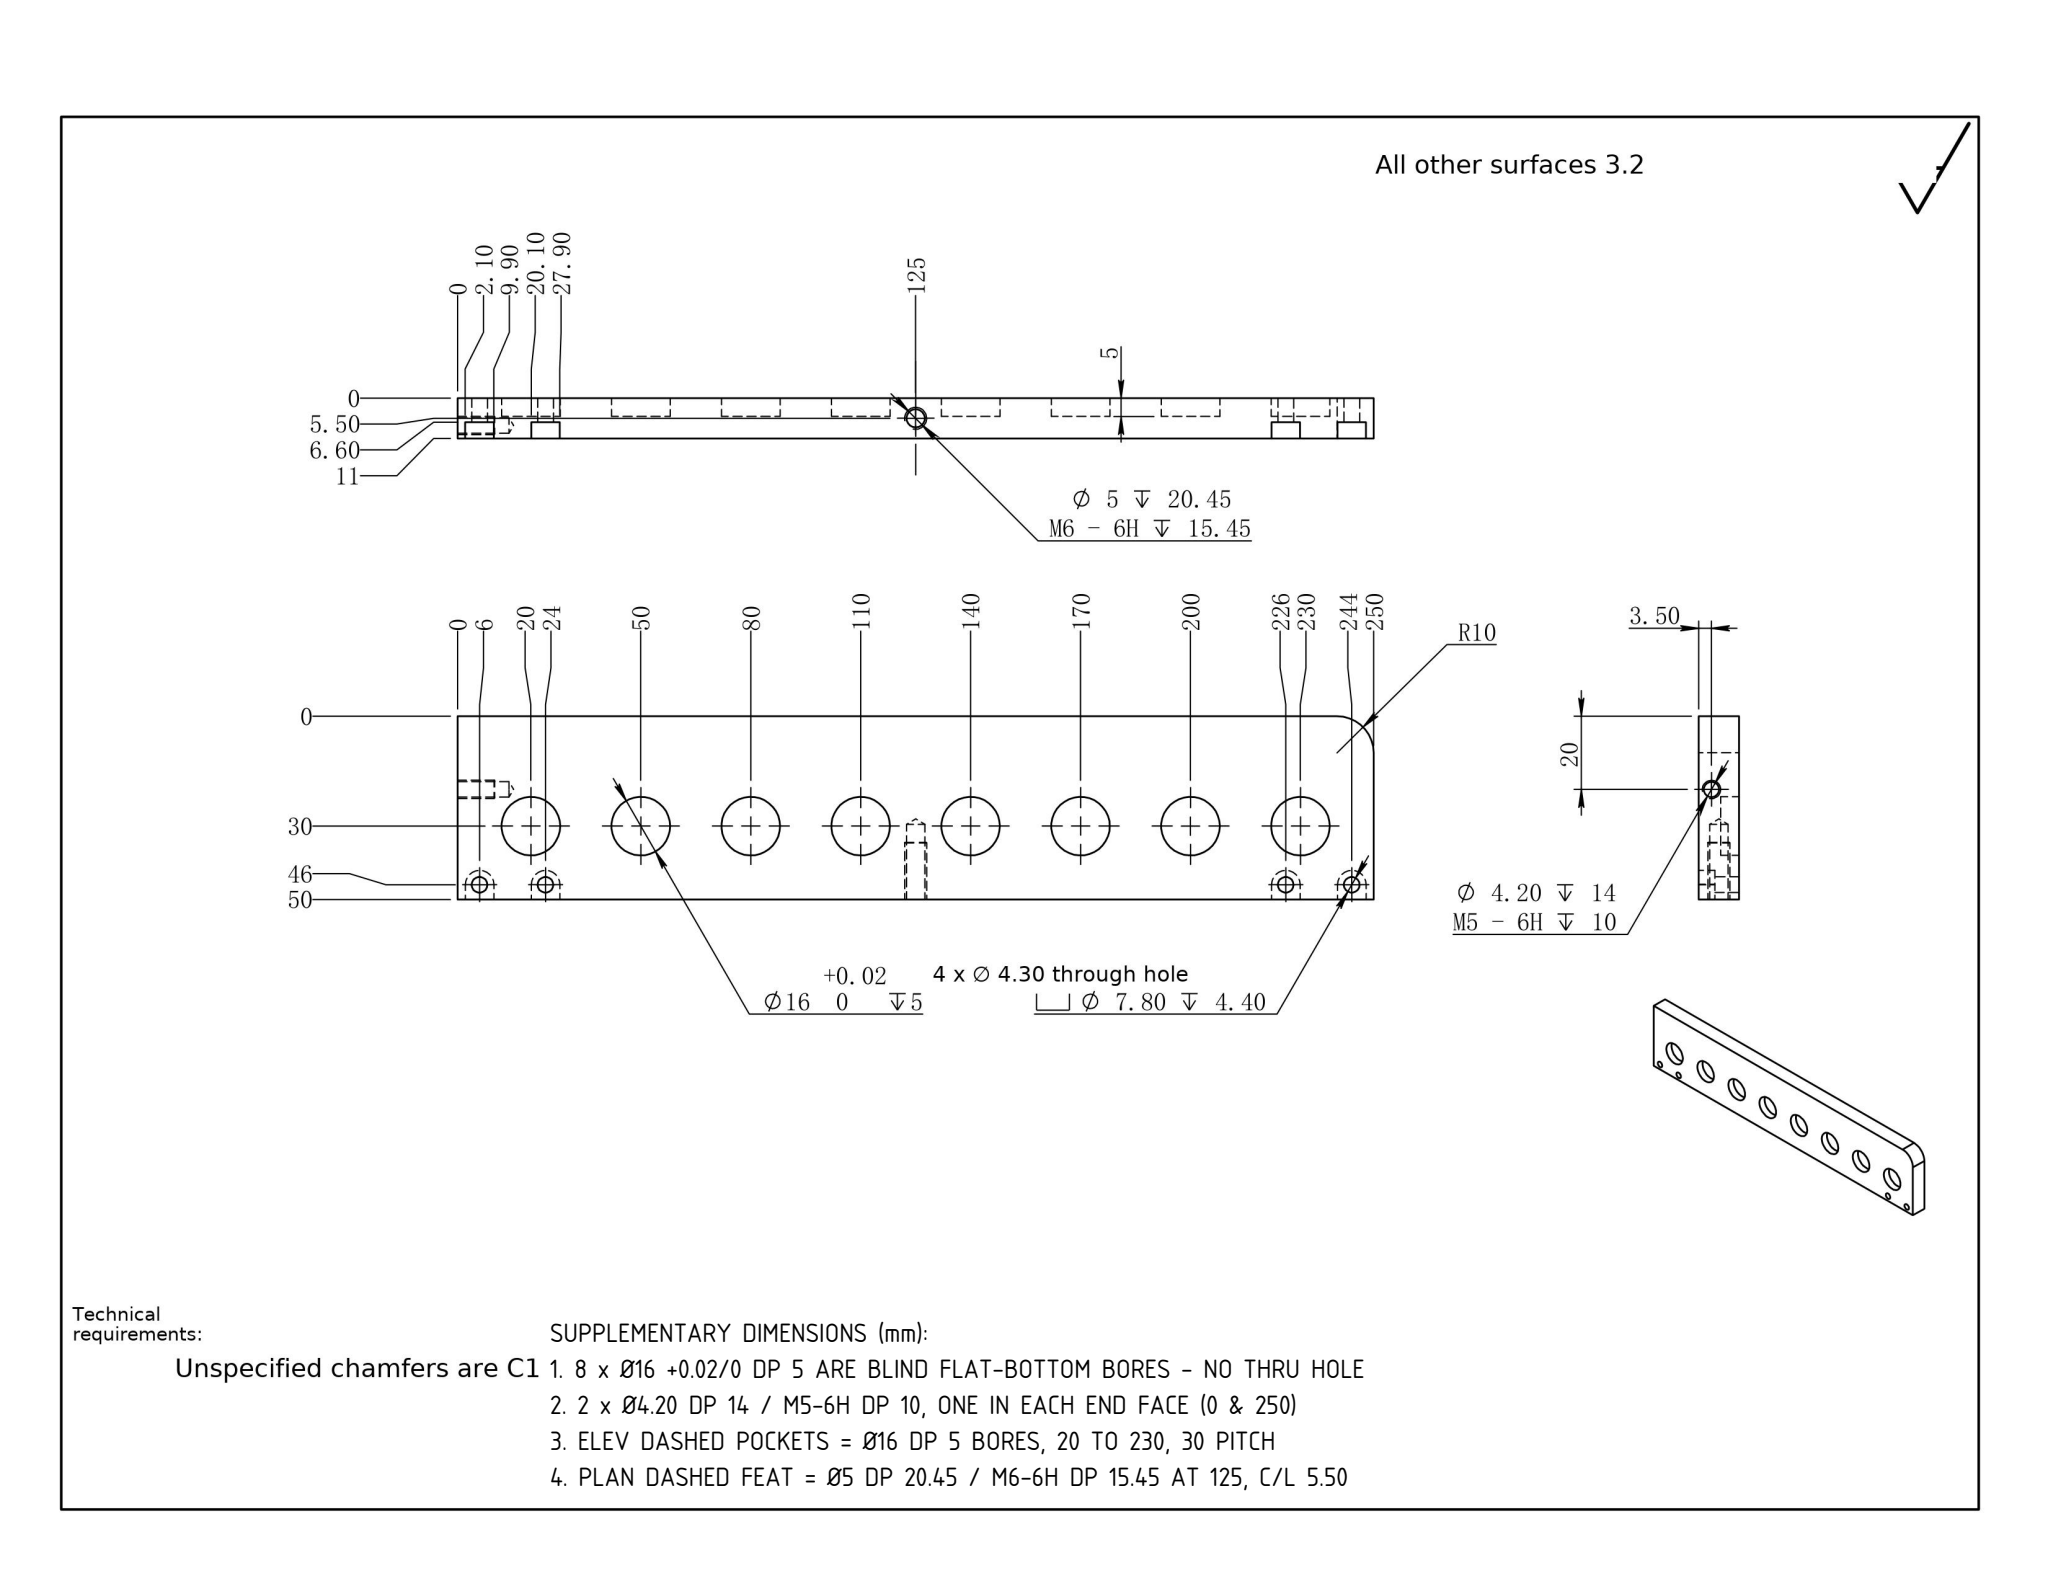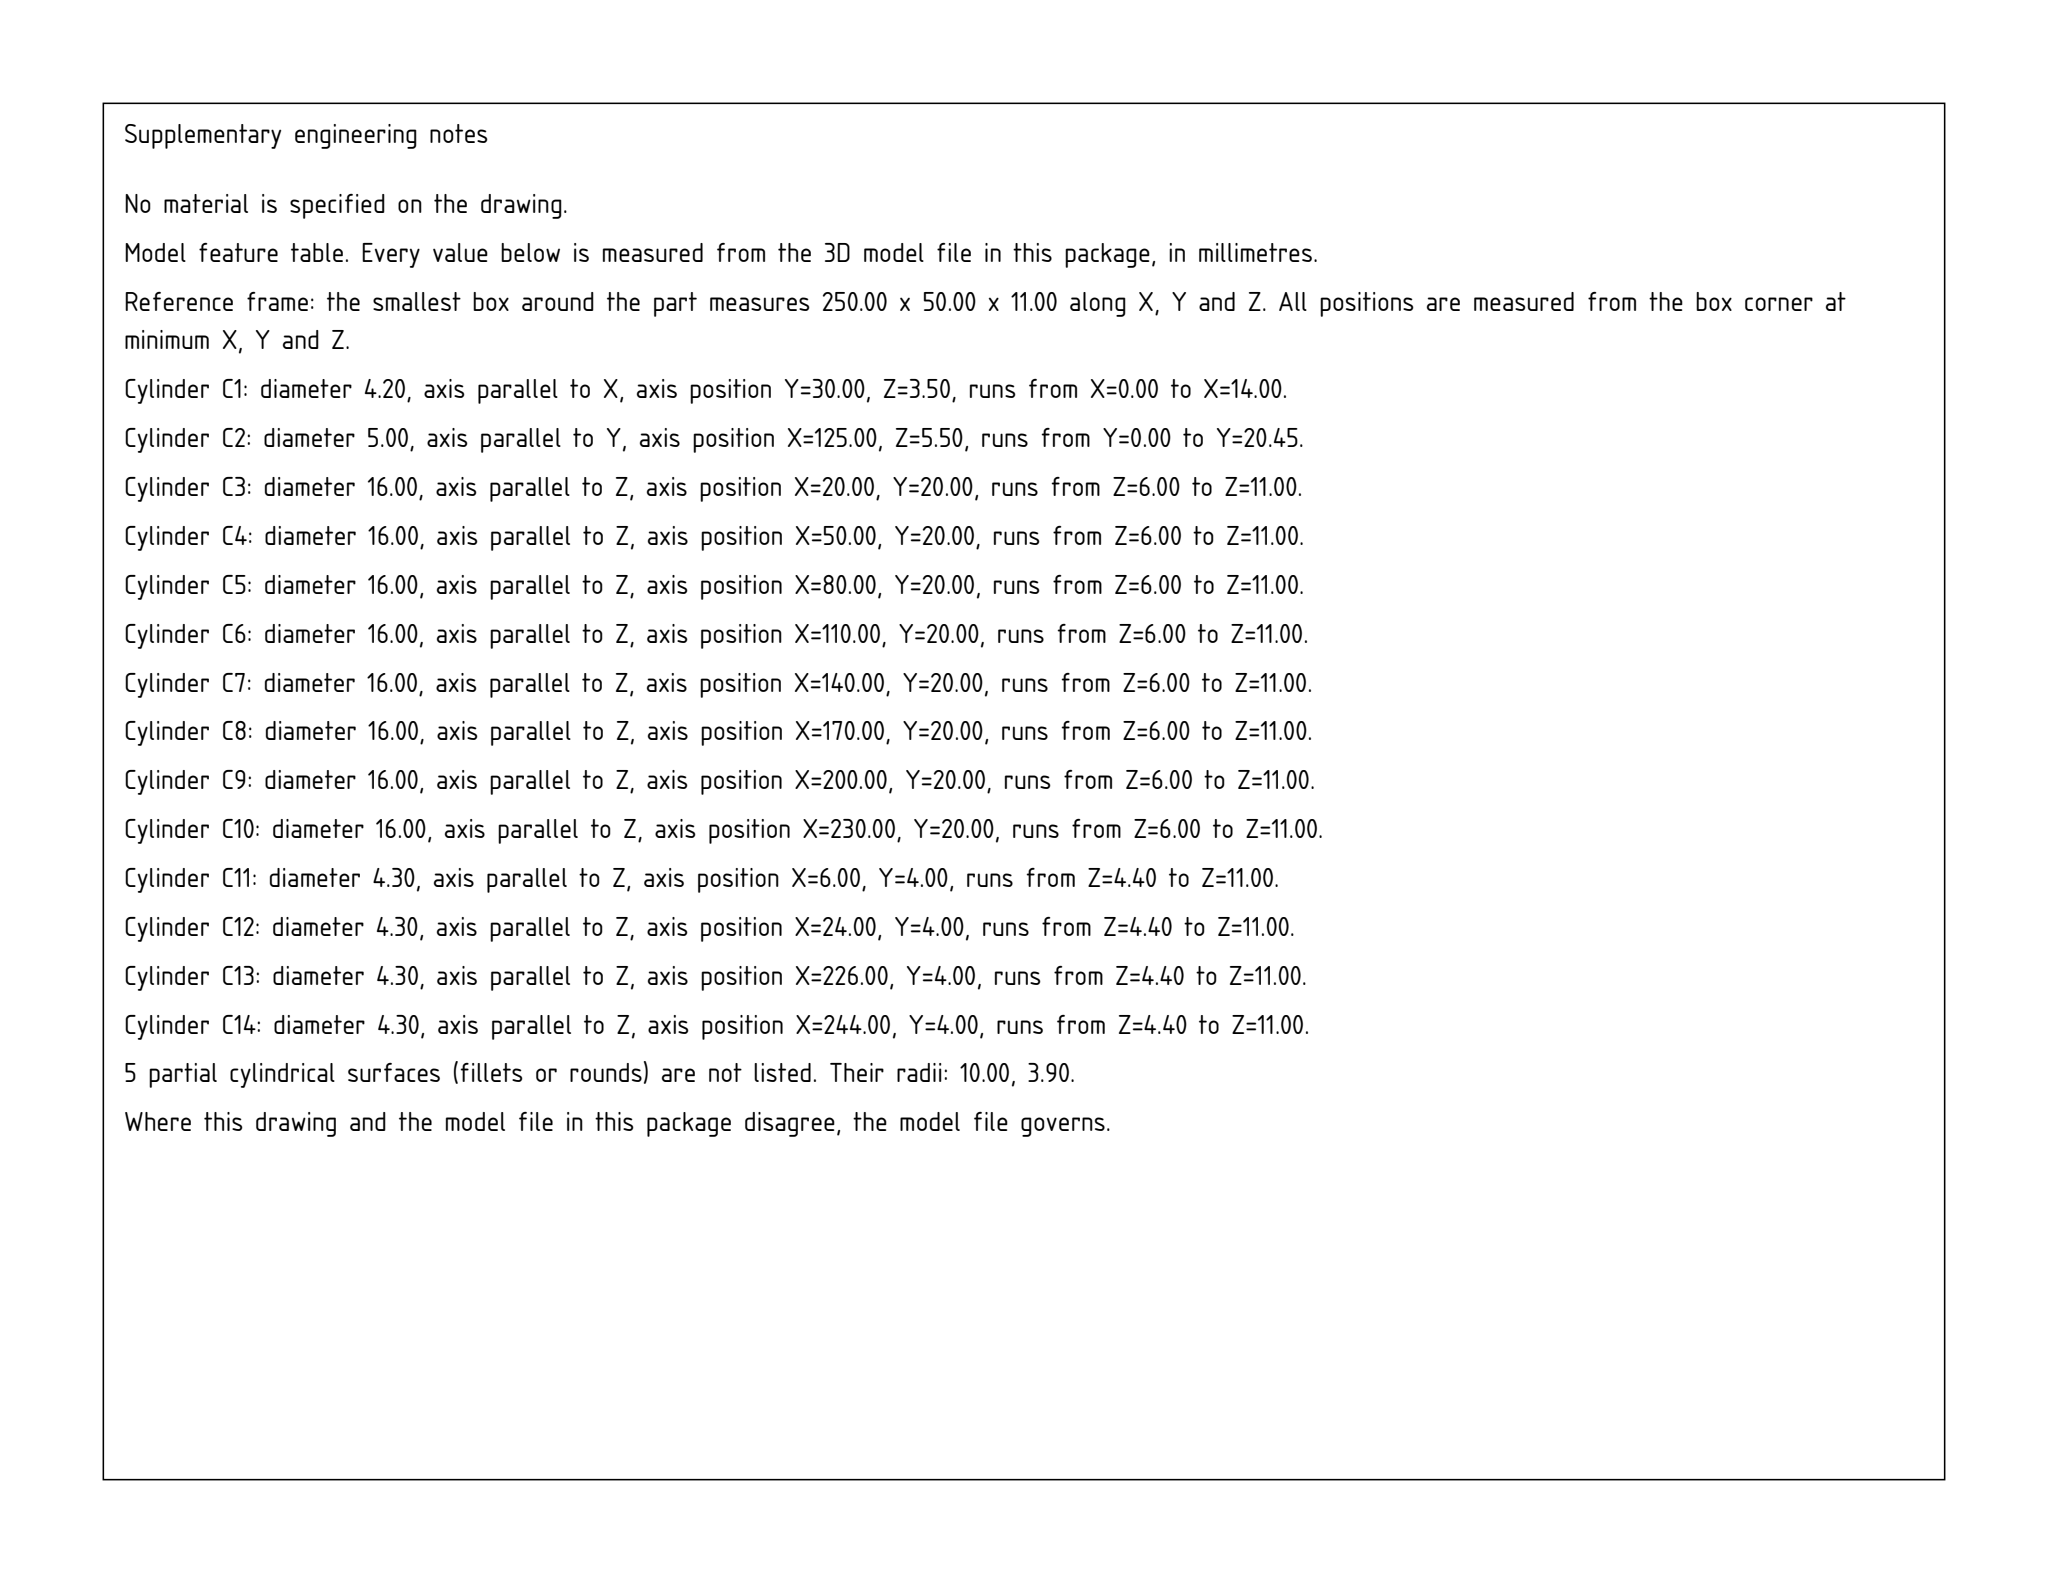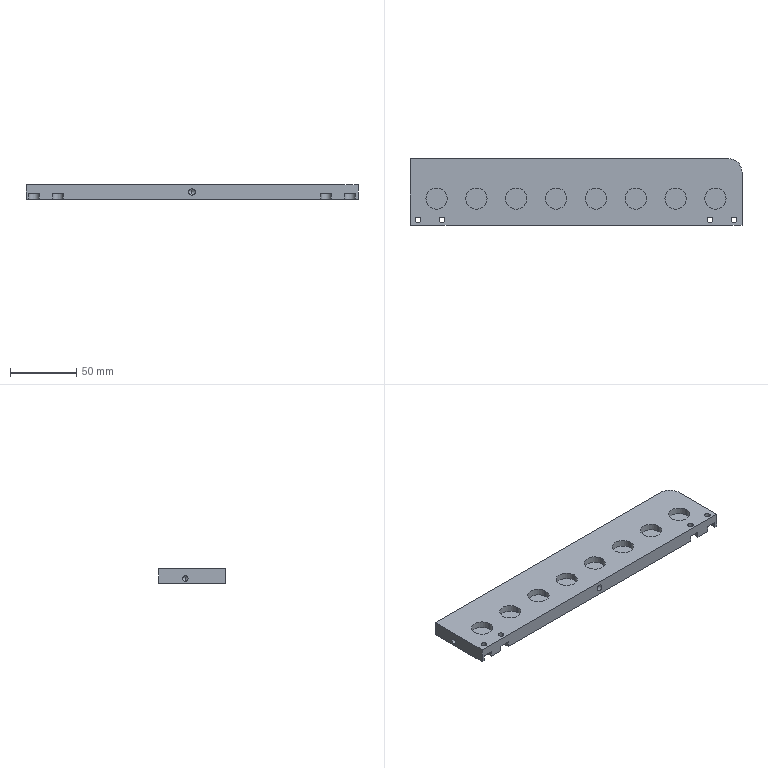Part | SolidWorks | mm | 1 solid | 63 faces | box 250 x 50 x 11 mm | volume 127257 mm3 | cylinder 33 | plane 26 | cone 4 | commonest cylinder face diameters 16 x16 4.3 x8 7.8 x4 4.2 x2 5 x2 20 x1
build123d program:
from build123d import *

# Parameters (mm, degrees)
SKETCH1_W                                       = 250
SKETCH1_H                                       = 50
BOSS_EXTRUDE1_DEPTH                             = 5.5
SKETCH2_R                                       = 8
CUT_EXTRUDE1_DEPTH                              = 5
LPATTERN1_COUNT                                 = 8
LPATTERN1_PITCH                                 = 30
FILLET4_R                                       = 10
M4_HEX_SOCKET_HEAD_CAP_SCREW_CBORE2_D           = 4.3
M4_HEX_SOCKET_HEAD_CAP_SCREW_CBORE2_CBORE_D     = 7.8
M4_HEX_SOCKET_HEAD_CAP_SCREW_CBORE2_CBORE_DEPTH = 4.4
CUT_EXTRUDE3_DEPTH                              = 128.646
M6_TAPPED_HOLE1_D                               = 5
M6_TAPPED_HOLE1_DEPTH                           = 20.45
M6_TAPPED_HOLE1_TIP                             = 1.502
M5_TAPPED_HOLE1_D                               = 4.2
M5_TAPPED_HOLE1_DEPTH                           = 14
M5_TAPPED_HOLE1_TIP                             = 1.262


with BuildPart() as part:
    # Sketch1 → Boss-Extrude1 (new, symmetric)
    with BuildSketch(Plane.XY):
        Rectangle(SKETCH1_W, SKETCH1_H)
    extrude(amount=BOSS_EXTRUDE1_DEPTH, both=True)

    # Sketch2 → Cut-Extrude1 (cut)
    with BuildSketch(Plane.XY.offset(5.5)):
        with Locations((105, -5)):
            Circle(SKETCH2_R)
    cut_extrude1 = extrude(amount=-CUT_EXTRUDE1_DEPTH, mode=Mode.SUBTRACT)

    # LPattern1: Cut-Extrude1 ×8
    with Locations(*[(-i * LPATTERN1_PITCH, 0, 0) for i in range(1, LPATTERN1_COUNT)]):
        add(cut_extrude1, mode=Mode.SUBTRACT)

    # Fillet4
    fillet4_edges = [part.edges().sort_by_distance(p)[0] for p in [
        (125, 25, 0),
    ]]
    fillet(fillet4_edges, radius=FILLET4_R)

    # M4 Hex Socket Head Cap Screw CBORE2 (through all)
    with Locations(Plane(origin=(0, 0, -5.5), x_dir=(-1, 0, 0), z_dir=(0, 0, -1))):
        with Locations((101, -21), (119, -21), (-119, -21), (-101, -21)):
            CounterBoreHole(M4_HEX_SOCKET_HEAD_CAP_SCREW_CBORE2_D / 2, M4_HEX_SOCKET_HEAD_CAP_SCREW_CBORE2_CBORE_D / 2, M4_HEX_SOCKET_HEAD_CAP_SCREW_CBORE2_CBORE_DEPTH)

    # Sketch8 → Cut-Extrude3 (cut, through all)
    with BuildSketch(Plane(origin=(0, 0, -1.1), x_dir=(-1, 0, 0), z_dir=(0, 0, -1))):
        with BuildLine():
            Line((-115.1, -21), (-115.1, -25))
            ThreePointArc((-115.1, -25), (-119, -28.9), (-122.9, -25))
            Line((-122.9, -25), (-122.9, -21))
            ThreePointArc((-122.9, -21), (-119, -17.1), (-115.1, -21))
        make_face()
        with BuildLine():
            Line((-97.1, -21), (-97.1, -25))
            ThreePointArc((-97.1, -25), (-101, -28.9), (-104.9, -25))
            Line((-104.9, -25), (-104.9, -21))
            ThreePointArc((-104.9, -21), (-101, -17.1), (-97.1, -21))
        make_face()
        with BuildLine():
            Line((104.9, -21), (104.9, -25))
            ThreePointArc((104.9, -25), (101, -28.9), (97.1, -25))
            Line((97.1, -25), (97.1, -21))
            ThreePointArc((97.1, -21), (101, -17.1), (104.9, -21))
        make_face()
        with BuildLine():
            Line((122.9, -21), (122.9, -25))
            ThreePointArc((122.9, -25), (119, -28.9), (115.1, -25))
            Line((115.1, -25), (115.1, -21))
            ThreePointArc((115.1, -21), (119, -17.1), (122.9, -21))
        make_face()
    extrude(amount=CUT_EXTRUDE3_DEPTH, mode=Mode.SUBTRACT)

    # M6 Tapped Hole1
    with Locations(Plane(origin=(0, -25, 0), x_dir=(-1, 0, 0), z_dir=(0, -1, 0))):
        with Locations((0, 0)):
            Hole(M6_TAPPED_HOLE1_D / 2, depth=M6_TAPPED_HOLE1_DEPTH)
            with Locations((0, 0, -(M6_TAPPED_HOLE1_DEPTH + M6_TAPPED_HOLE1_TIP / 2))):  # 118° drill point
                Cone(0, M6_TAPPED_HOLE1_D / 2, M6_TAPPED_HOLE1_TIP, mode=Mode.SUBTRACT)

    # M5 Tapped Hole1
    with Locations(Plane.ZY.offset(125)):
        with Locations((-2, 5)):
            Hole(M5_TAPPED_HOLE1_D / 2, depth=M5_TAPPED_HOLE1_DEPTH)
            with Locations((0, 0, -(M5_TAPPED_HOLE1_DEPTH + M5_TAPPED_HOLE1_TIP / 2))):  # 118° drill point
                Cone(0, M5_TAPPED_HOLE1_D / 2, M5_TAPPED_HOLE1_TIP, mode=Mode.SUBTRACT)


solid = part.part